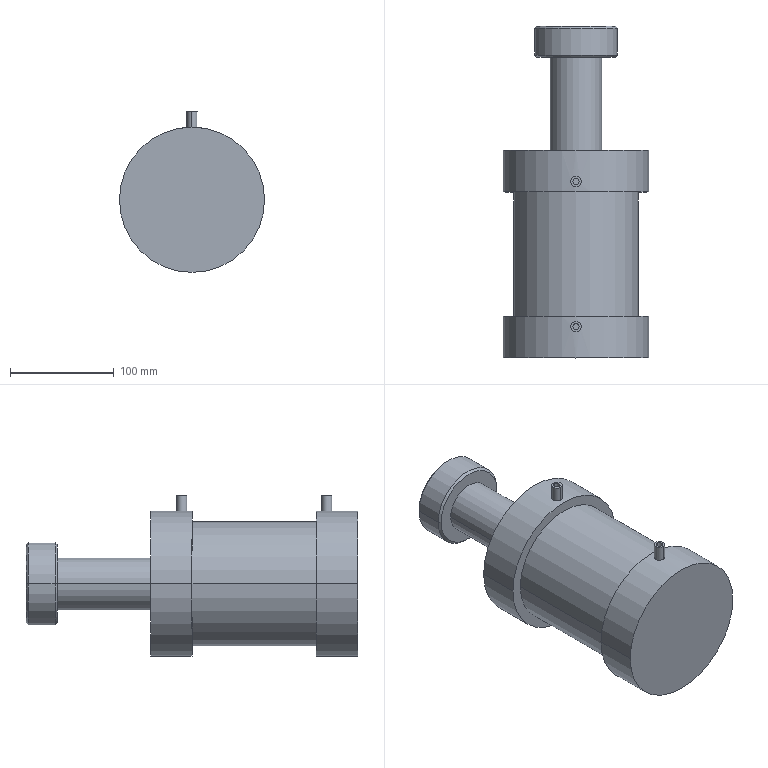Component | SolidWorks | HydraulicCylinderB-1 | 3 solids | 38 faces | box 140 x 320 x 155 mm | volume 2912748 mm3 | cylinder 22 | plane 12 | cone 4 | commonest cylinder face diameters 10 x8 140 x4 6 x4 80 x2 120 x2 50 x2 | material 45
build123d program:
from build123d import *

# Parameters (mm, degrees)
SKETCH2_2_R           = 40
BOSS_EXTRUDE1_DEPTH   = 30
CHAMFER1_SIZE         = 2
SKETCH2_R             = 5
CUT_EXTRUDE2_DEPTH    = 75
SKETCH4_R             = 5
SKETCH4_R_2           = 3
BOSS_EXTRUDE3_DEPTH   = 85
BOSS_EXTRUDE3_2_DEPTH = 85


with BuildPart() as part:
    # Sketch1 → Revolve1 (revolve)
    with BuildSketch(Plane.XY, mode=Mode.PRIVATE) as revolve1_sk:
        Polygon((0, 0), (0, 25), (90, 25), (90, 70), (130, 70), (130, 60), (250, 60), (250, 70), (290, 70), (290, 0), align=None)
    revolve(revolve1_sk.sketch.rotate(Axis((0, 0, 0), (1, 0, 0)), 180), axis=Axis((0, 0, 0), (1, 0, 0)))

    # Sketch2_2 → Boss-Extrude1 (add)
    with BuildSketch(Plane.ZY):
        with Locations(Location((0, 0, 0), (0, 0, 270))):
            Circle(SKETCH2_2_R)
    extrude(amount=BOSS_EXTRUDE1_DEPTH)

    # Chamfer1
    chamfer1_edges = [part.edges().sort_by_distance(p)[0] for p in [
        (0, 40, 0),
        (-30, 40, 0),
    ]]
    chamfer(chamfer1_edges, length=CHAMFER1_SIZE)

    # Sketch2 → Cut-Extrude2 (cut)
    with BuildSketch(Plane.XY):
        with Locations(Location((120, 0, 0), (0, 0, 180))):
            Circle(SKETCH2_R)
        with Locations(Location((260, 0, 0), (0, 0, 180))):
            Circle(SKETCH2_R)
    extrude(amount=CUT_EXTRUDE2_DEPTH, mode=Mode.SUBTRACT)


with BuildPart() as body_2:
    # Sketch4 → Boss-Extrude3 (new body)
    with BuildSketch(Plane.XY):
        with Locations((120, 0)):
            Circle(SKETCH4_R)
        with Locations((120, 0)):
            Circle(SKETCH4_R_2, mode=Mode.SUBTRACT)
    extrude(amount=BOSS_EXTRUDE3_DEPTH)


with BuildPart() as body_3:
    # Sketch4 → Boss-Extrude3 2 (new body)
    with BuildSketch(Plane.XY):
        with Locations((260, 0)):
            Circle(SKETCH4_R)
        with Locations((260, 0)):
            Circle(SKETCH4_R_2, mode=Mode.SUBTRACT)
    extrude(amount=BOSS_EXTRUDE3_2_DEPTH)


solid = Compound([part.part, body_2.part, body_3.part])

# Placed as in the assembly
solid = solid.moved(Location((-90.812, -41.571, 100), (0, 0, -90)))